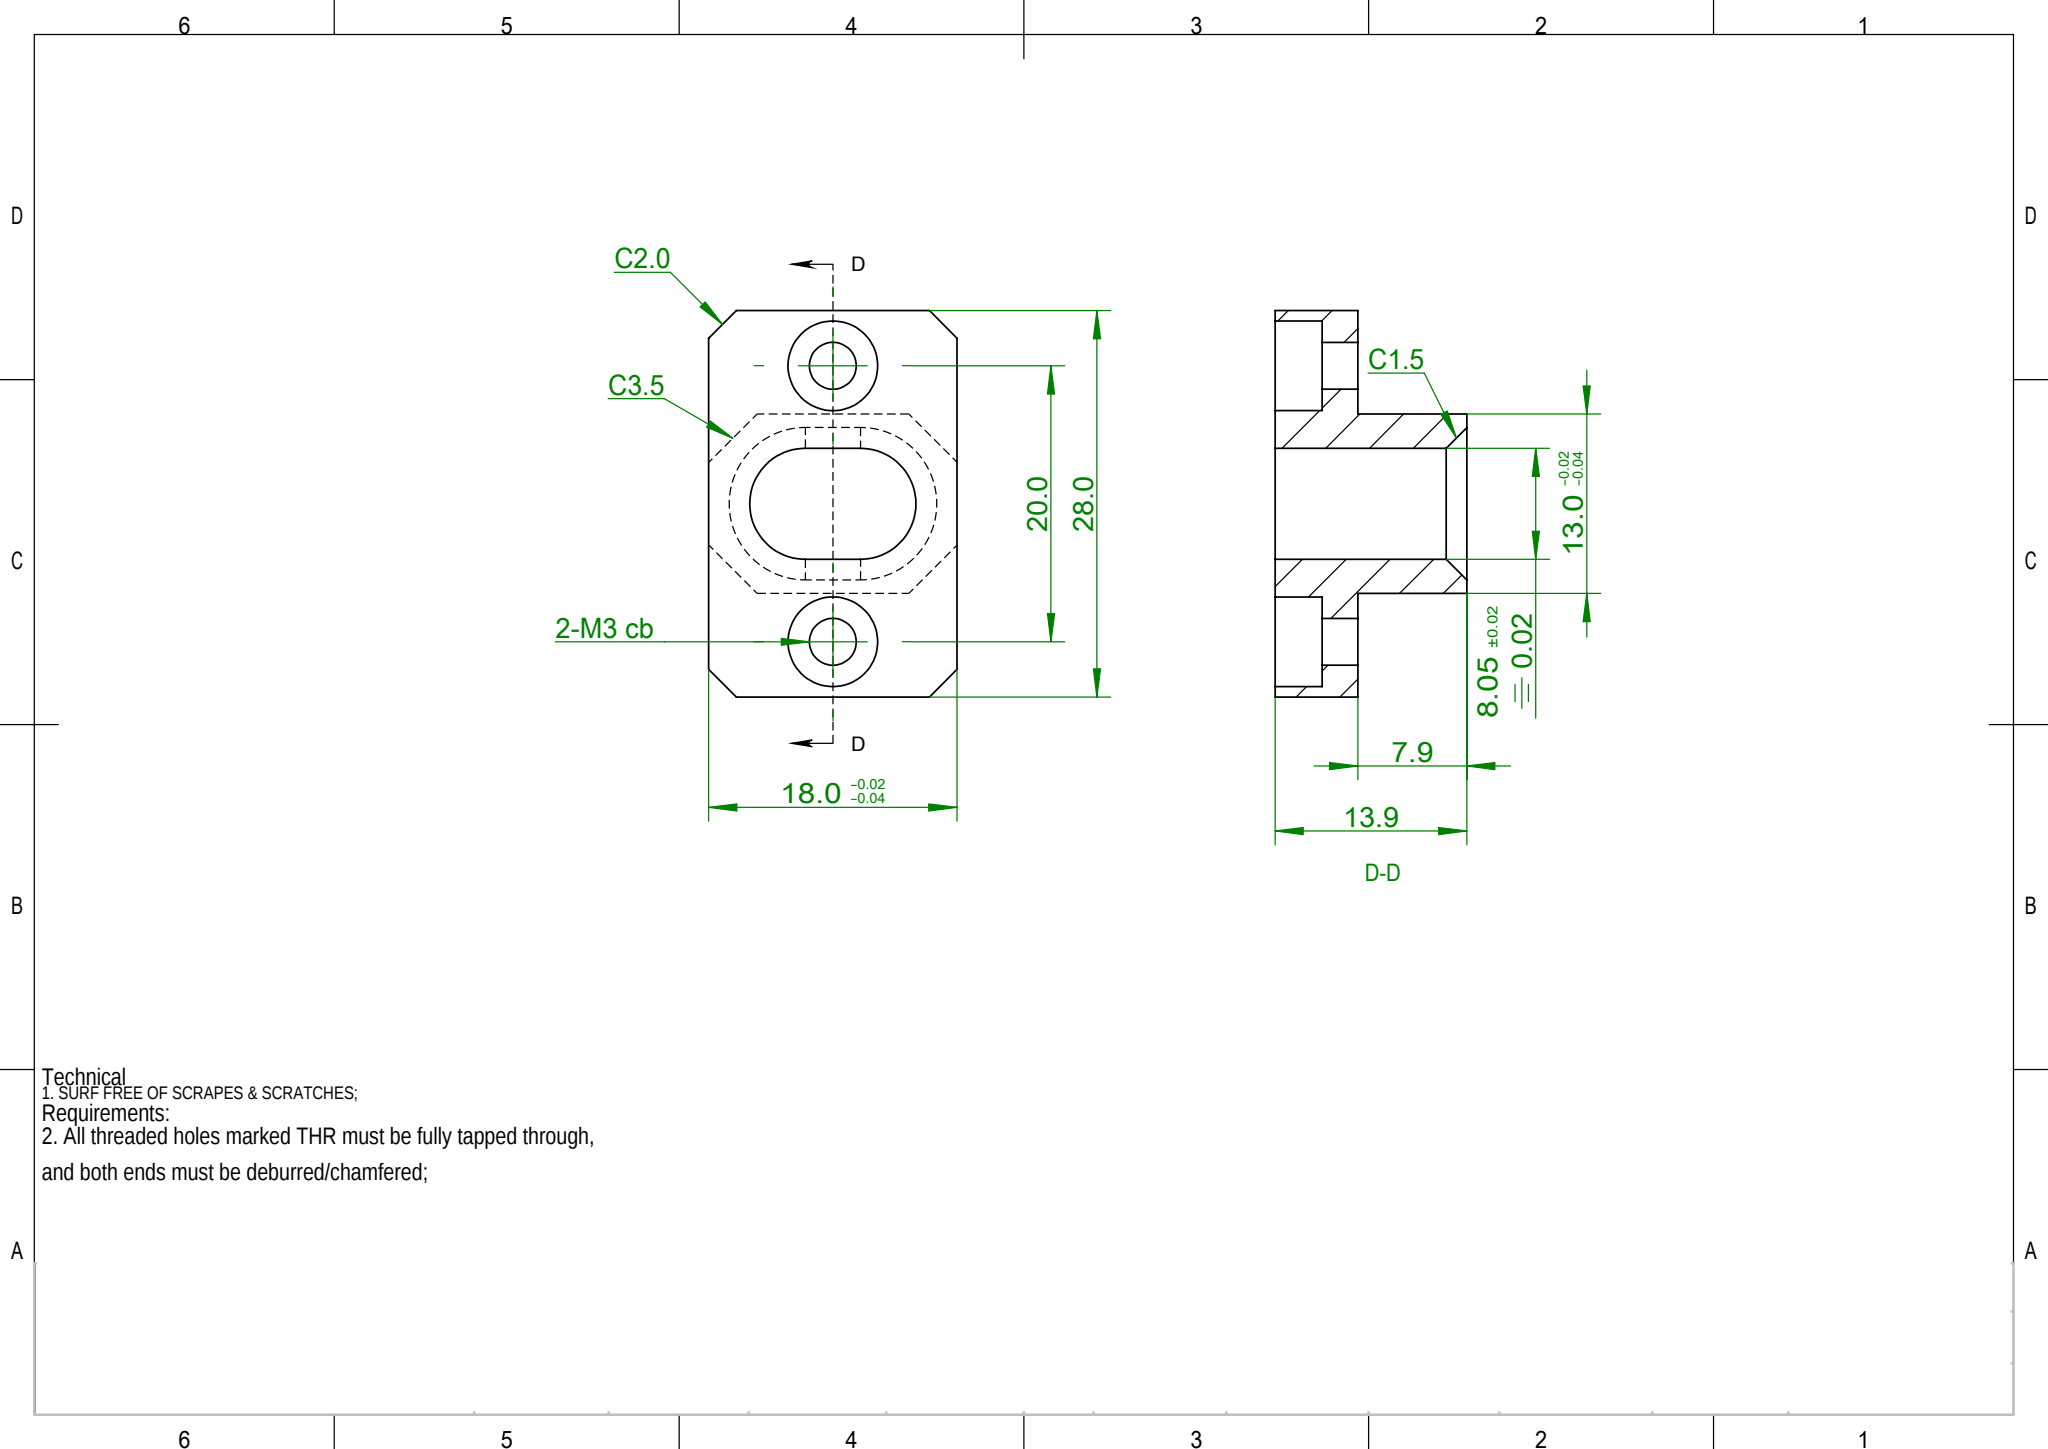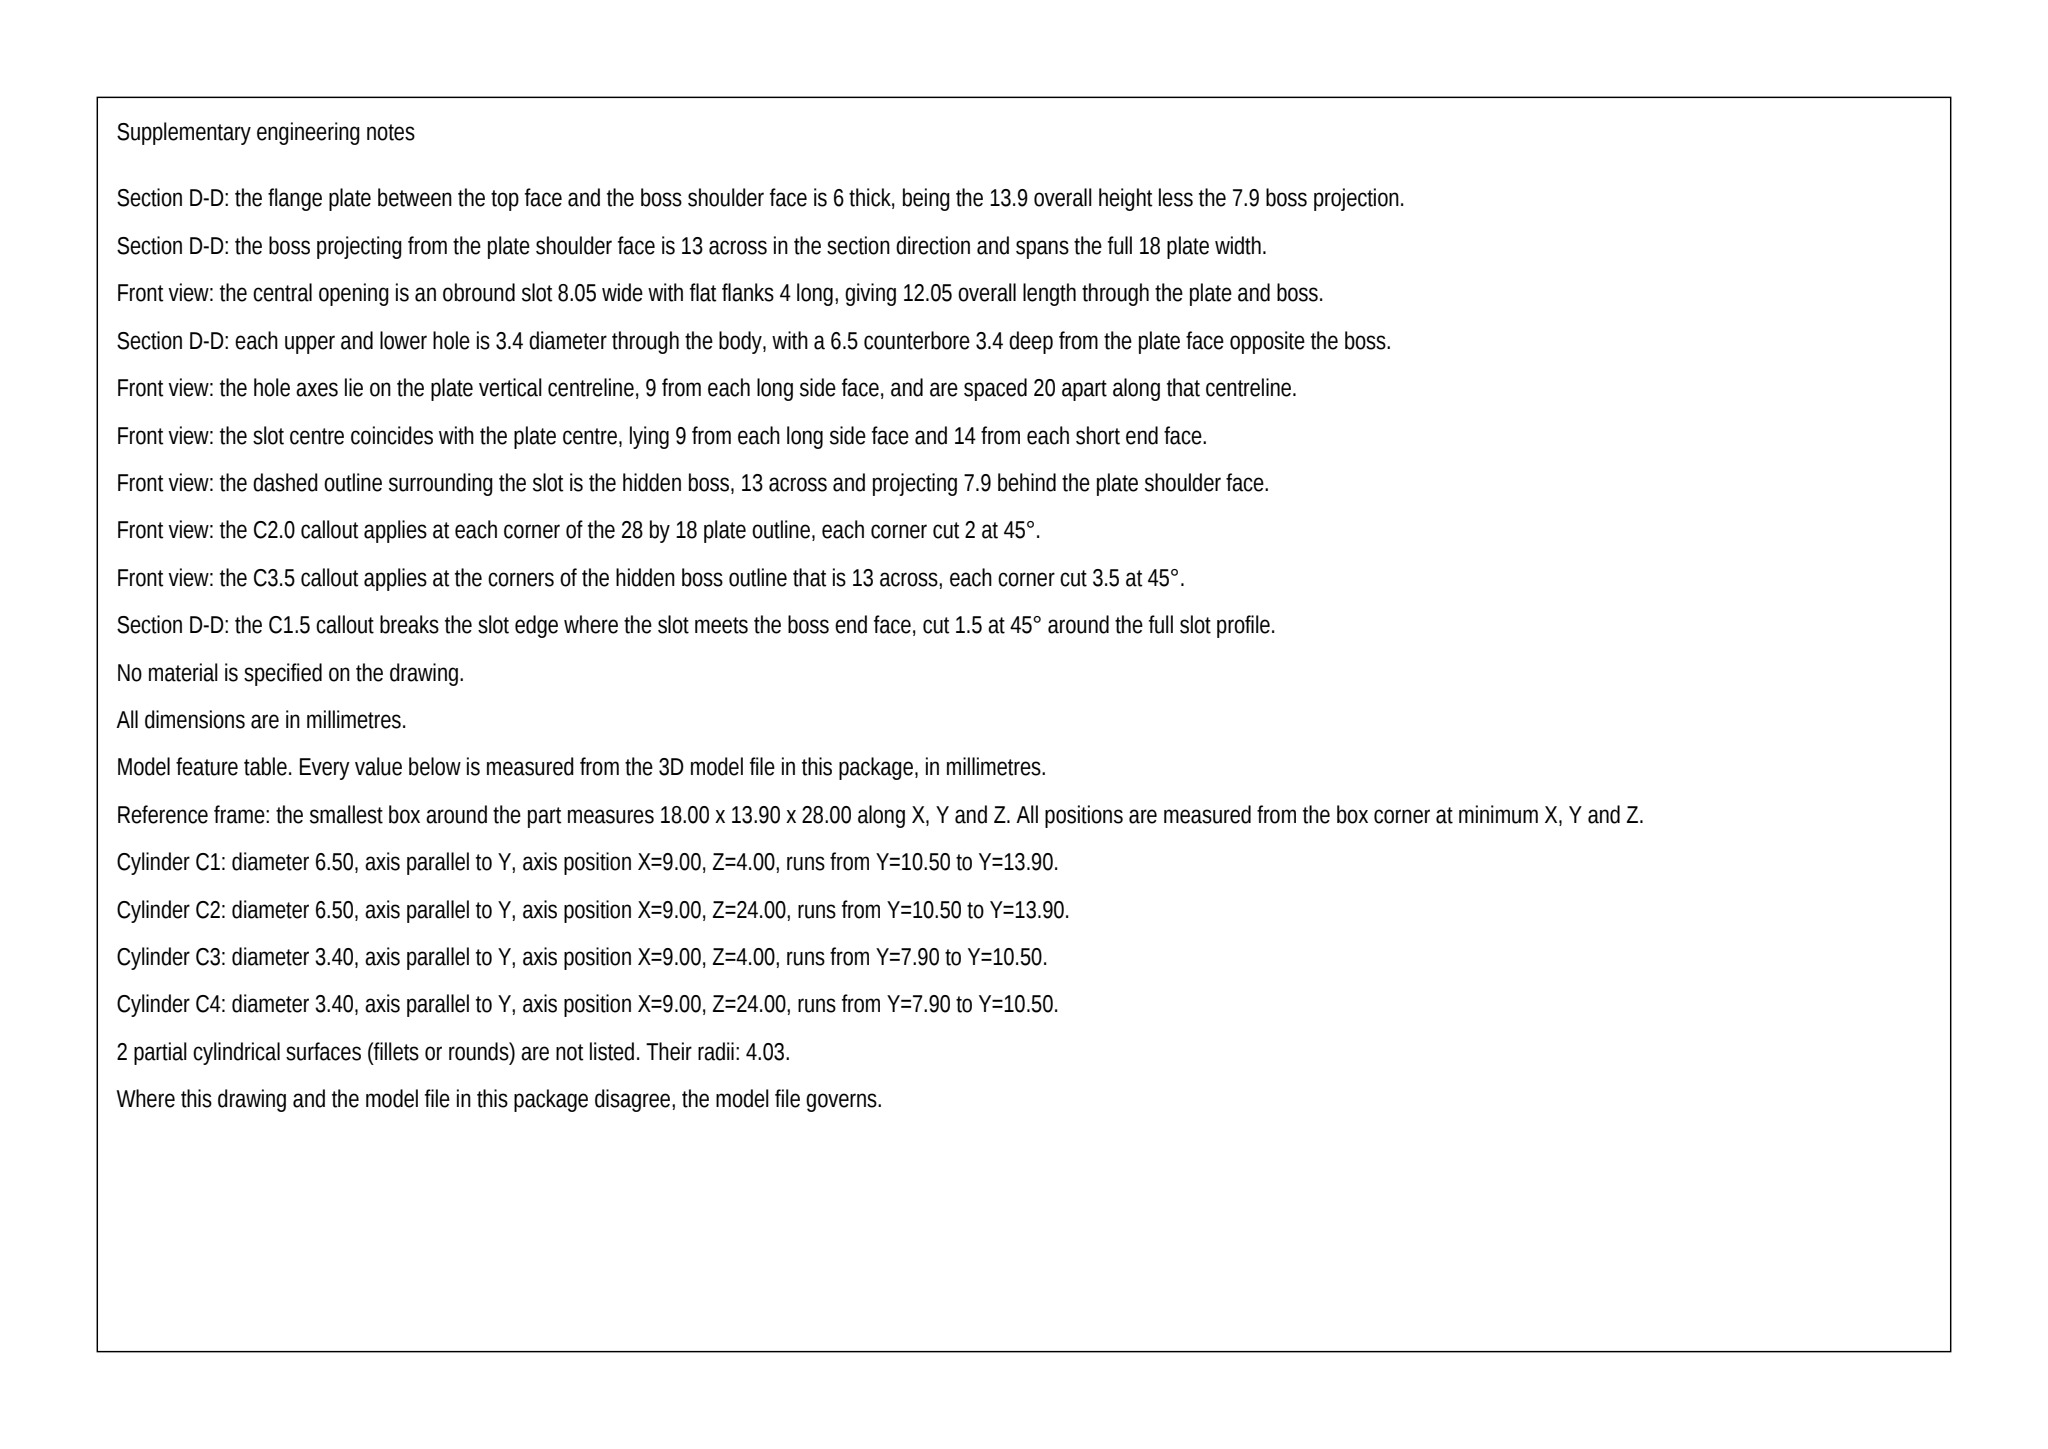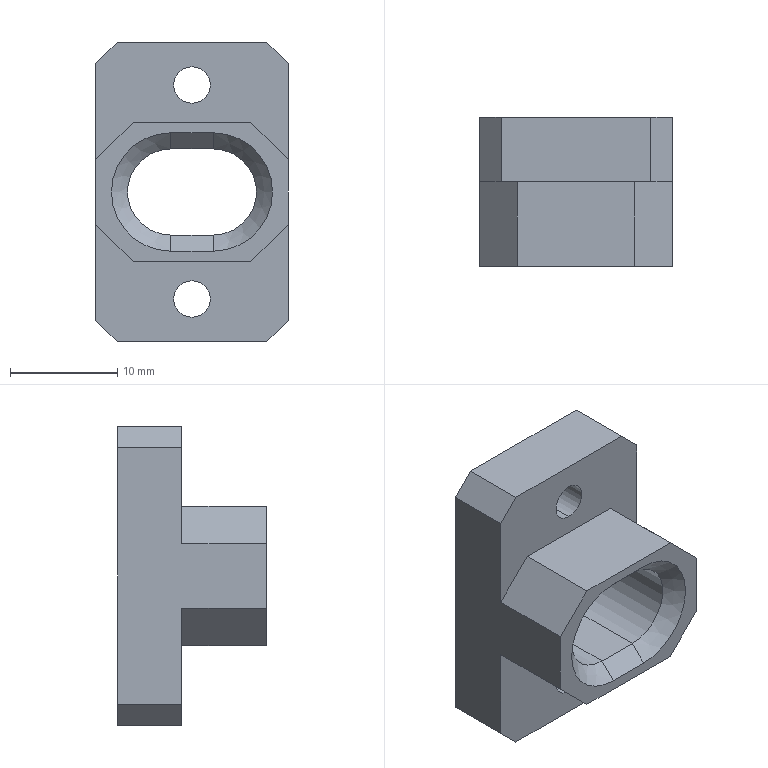Part | SolidWorks | mm | 1 solid | 36 faces | box 18 x 13.9 x 28 mm | volume 3162 mm3 | plane 24 | cylinder 10 | cone 2 | commonest cylinder face diameters 6.5 x4 3.4 x4 8.05 x2
Drawing notes:
BOSS: 18.0 WIDE (FULL) X 13.0 HIGH CTRD, PROJ 7.9 FROM FLANGE | from the solid: X planes only at 0.0 and 18.0 (boss full plate width); Z planes 7.5/20.5 = 13.0 ctrd on 28.0; Y planes 0/7.9/13.9 -> boss 7.9 deep, flange 6.0
CTR BORE: OBROUND 8.05 WIDE X 12.05 LG THRU, 2X R4.025 ON 4.0 | from the solid: Ø8.05 cyls, axis Y, at x=7.0 and x=11.0, z=14.0; 4.0 + 8.05 = 12.05 overall
2X Ø3.4 THRU, CBORE Ø6.5 DP 3.4; 20.0 APART ON CL OF 18.0 | from the solid: Ø3.4 y-cyls at (9.0,4.0) and (9.0,24.0) L=2.6; Ø6.5 cbores same axes L=3.4; 24.0-4.0=20.0; x=9.0=18.0/2
DEL 2-M3 CB: HOLES ARE Ø3.4 CLEARANCE W/ CBORE Ø6.5 DP 3.4 | from the solid: No thread geometry; bores are plain Ø3.4 (2.6 lg) + Ø6.5 (3.4 lg) = 6.0 flange thk
CTR BORE Ø8.05 ±0.02; MOVE 0.02 TOL FRAME CLEAR OF DIM TEXT | from the solid: Ø8.05 cylinders, length 12.4, 90° chamfer cones ref dia 8.05
build123d program:
from build123d import *

# Parameters (mm, degrees)
SKETCH1_W                                       = 18
SKETCH1_H                                       = 13
BOSS_EXTRUDE1_DEPTH                             = 7.9
SKETCH2_W                                       = 18
SKETCH2_H                                       = 28
BOSS_EXTRUDE2_DEPTH                             = 5
M3_HEX_SOCKET_HEAD_CAP_SCREW_CBORE1_D           = 3.4
M3_HEX_SOCKET_HEAD_CAP_SCREW_CBORE1_CBORE_D     = 6.5
M3_HEX_SOCKET_HEAD_CAP_SCREW_CBORE1_CBORE_DEPTH = 3.4
CHAMFER1_SIZE                                   = 2
CUT_EXTRUDE1_DEPTH                              = 111
CHAMFER2_SIZE                                   = 1.5
CHAMFER3_SIZE                                   = 3.5
MOVE_FACE1_BY                                   = 1
MOVE_FACE1_2_BY                                 = 1
MOVE_FACE1_3_BY                                 = 1


with BuildPart() as part:
    # Sketch1 → Boss-Extrude1 (new body)
    with BuildSketch(Plane(origin=(0, 0, 0), x_dir=(1, 0, 0), z_dir=(0, 1, 0))):
        Rectangle(SKETCH1_W, SKETCH1_H)
    extrude(amount=-BOSS_EXTRUDE1_DEPTH)

    # Sketch2 → Boss-Extrude2 (add)
    with BuildSketch(Plane(origin=(0, 0, 0), x_dir=(1, 0, 0), z_dir=(0, 1, 0))):
        Rectangle(SKETCH2_W, SKETCH2_H)
    extrude(amount=BOSS_EXTRUDE2_DEPTH)

    # M3 Hex Socket Head Cap Screw CBORE1 (through all)
    with Locations(Plane(origin=(0, 5, 0), x_dir=(1, 0, 0), z_dir=(0, 1, 0))):
        with Locations((0, 10), (0, -10)):
            CounterBoreHole(M3_HEX_SOCKET_HEAD_CAP_SCREW_CBORE1_D / 2, M3_HEX_SOCKET_HEAD_CAP_SCREW_CBORE1_CBORE_D / 2, M3_HEX_SOCKET_HEAD_CAP_SCREW_CBORE1_CBORE_DEPTH)

    # Chamfer1
    chamfer1_edges = [part.edges().sort_by_distance(p)[0] for p in [
        (9, 2.5, 14),
        (9, 2.5, -14),
        (-9, 2.5, -14),
        (-9, 2.5, 14),
    ]]
    chamfer(chamfer1_edges, length=CHAMFER1_SIZE)

    # Sketch5 → Cut-Extrude1 (cut)
    with BuildSketch(Plane(origin=(0, 5, 0), x_dir=(1, 0, 0), z_dir=(0, 1, 0))):
        with BuildLine():
            Line((-2, 4.025), (2, 4.025))
            ThreePointArc((2, 4.025), (6.025, 0), (2, -4.025))
            Line((2, -4.025), (-2, -4.025))
            ThreePointArc((-2, -4.025), (-6.025, 0), (-2, 4.025))
        make_face()
    extrude(amount=-CUT_EXTRUDE1_DEPTH, mode=Mode.SUBTRACT)

    # Chamfer2
    chamfer2_edges = [part.edges().sort_by_distance(p)[0] for p in [
        (-6.025, -7.9, 0),
        (0, -7.9, -4.025),
        (6.025, -7.9, 0),
        (0, -7.9, 4.025),
    ]]
    chamfer(chamfer2_edges, length=CHAMFER2_SIZE)

    # Chamfer3
    chamfer3_edges = [part.edges().sort_by_distance(p)[0] for p in [
        (-9, -3.95, -6.5),
        (9, -3.95, -6.5),
        (9, -3.95, 6.5),
        (-9, -3.95, 6.5),
    ]]
    chamfer(chamfer3_edges, length=CHAMFER3_SIZE)

    # Move Face1: a face moved outward by 1.0
    extrude(part.faces().sort_by_distance((0, 1.6, 12.6))[0], amount=MOVE_FACE1_BY, dir=(0, 1, 0))

    # Move Face1 2: a face moved outward by 1.0
    extrude(part.faces().sort_by_distance((0, 1.6, -7.4))[0], amount=MOVE_FACE1_2_BY, dir=(0, 1, 0))

    # Move Face1 3: a face moved outward by 1.0
    extrude(part.faces().sort_by_distance((4.5, 5, 7))[0], amount=MOVE_FACE1_3_BY, dir=(0, 1, 0))


solid = part.part